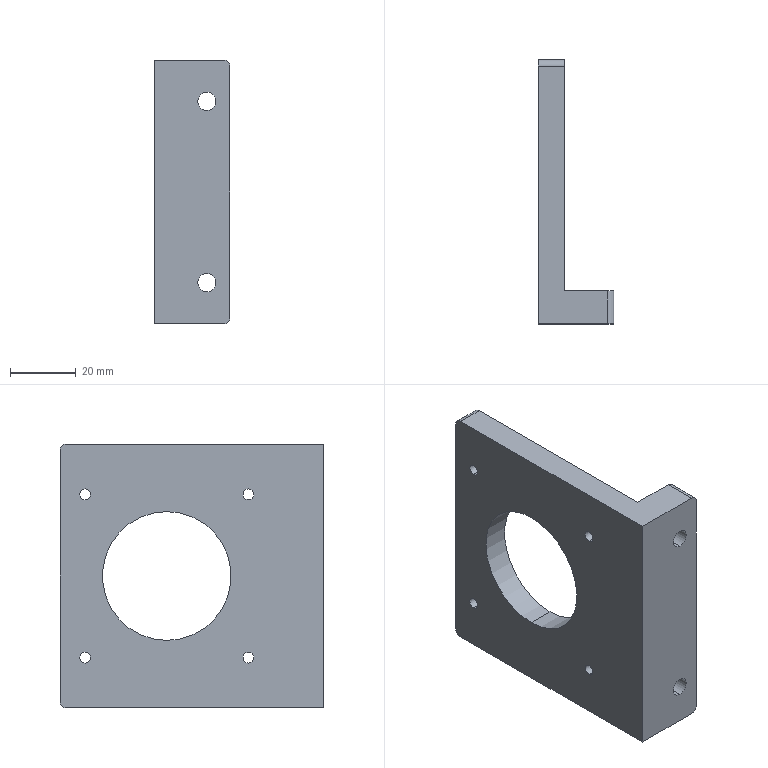Component | SolidWorks | ZHDJ-G003-1 | 1 solid | 32 faces | box 23 x 80 x 80 mm | volume 52239 mm3 | cylinder 22 | plane 10 | commonest cylinder face diameters 3.3 x8 10 x4 5.5 x4 4 x4 39 x2
build123d program:
from build123d import *

# Parameters (mm, degrees)
SKETCH1_W             = 80
SKETCH1_H             = 80
BOSS_EXTRUDE1_DEPTH   = 4
SKETCH2_W             = 80
SKETCH2_H             = 10
BOSS_EXTRUDE2_DEPTH   = 15
SKETCH3_R             = 19.5
CUT_EXTRUDE1_DEPTH    = 20
FILLET1_R             = 2
M4_TAPPED_HOLE1_D     = 3.3
M4_TAPPED_HOLE1_DEPTH = 11.5
M4_TAPPED_HOLE1_TIP   = 0.9914


with BuildPart() as part:
    # Sketch1 → Boss-Extrude1 (new, symmetric)
    with BuildSketch(Plane(origin=(0, 0, 0), x_dir=(0, 0, -1), z_dir=(1, 0, 0))):
        Rectangle(SKETCH1_W, SKETCH1_H)
    extrude(amount=BOSS_EXTRUDE1_DEPTH, both=True)

    # Sketch2 → Boss-Extrude2 (add)
    with BuildSketch(Plane(origin=(4, 0, 0), x_dir=(0, 0, -1), z_dir=(1, 0, 0))):
        with Locations((0, 35)):
            Rectangle(SKETCH2_W, SKETCH2_H)
    extrude(amount=BOSS_EXTRUDE2_DEPTH)

    # Sketch3 → Cut-Extrude1 (cut)
    with BuildSketch(Plane.ZY.offset(4)):
        with Locations((0, -7.641)):
            Circle(SKETCH3_R)
    extrude(amount=-CUT_EXTRUDE1_DEPTH, mode=Mode.SUBTRACT)

    # Fillet1
    fillet1_edges = [part.edges().sort_by_distance(p)[0] for p in [
        (19, 35, 40),
        (19, 35, -40),
        (0, -40, -40),
        (0, -40, 40),
    ]]
    fillet(fillet1_edges, radius=FILLET1_R)

    # Sketch4 → Hole Size _According to_ Type 1 of Hexag (revolve, cut)
    with BuildSketch(Plane(origin=(12, 30, -27.5), x_dir=(0, 0, -1), z_dir=(1, 0, 0))):
        Polygon((0, 0), (0, 15.652), (2.75, 14), (2.75, 5.7), (5, 5.7), (5, 0), align=None)
    hole_size_according_to_type_1_of_hexag = revolve(axis=Axis((12, 23.65, -27.5), (0, 1, 0)), mode=Mode.SUBTRACT)

    # Mirror1: Hole Size _According to_ Type 1 of Hexag across plane
    add(hole_size_according_to_type_1_of_hexag.mirror(Plane.XY), mode=Mode.SUBTRACT)

    # M4 Tapped Hole1
    with Locations(Plane(origin=(4, 17.108, 24.749), x_dir=(0, 0, 1), z_dir=(1, 0, 0))):
        with Locations((0, 0), (-49.497, 0), (-49.497, 49.497), (0, 49.497)):
            Hole(M4_TAPPED_HOLE1_D / 2, depth=M4_TAPPED_HOLE1_DEPTH)
            with Locations((0, 0, -(M4_TAPPED_HOLE1_DEPTH + M4_TAPPED_HOLE1_TIP / 2))):  # 118° drill point
                Cone(0, M4_TAPPED_HOLE1_D / 2, M4_TAPPED_HOLE1_TIP, mode=Mode.SUBTRACT)


solid = part.part

# Placed as in the assembly
solid = solid.moved(Location((-10, -107.5, 124.987), (180, 0, 0)))
STEP:
#1=COLOUR_RGB('',0.7922,0.8196,0.9333);
#2=FILL_AREA_STYLE_COLOUR('',#1);
#3=FILL_AREA_STYLE('',(#2));
#4=SURFACE_STYLE_FILL_AREA(#3);
#5=SURFACE_SIDE_STYLE('',(#4));
#6=SURFACE_STYLE_USAGE(.BOTH.,#5);
#7=PRESENTATION_STYLE_ASSIGNMENT((#6));
#8=CARTESIAN_POINT('',(-0.5512,-4.906,3.881));
#9=VERTEX_POINT('',#8);
#10=CARTESIAN_POINT('',(-0.5512,-4.906,4.011));
#11=VERTEX_POINT('',#10);
#12=CARTESIAN_POINT('',(-0.5512,-4.906,3.946));
#13=DIRECTION('',(1.,-0.,-0.));
#14=DIRECTION('',(0.,0.,1.));
#15=AXIS2_PLACEMENT_3D('',#12,#13,#14);
#16=CIRCLE('',#15,0.06496);
#17=EDGE_CURVE('',#9,#11,#16,.T.);
#18=ORIENTED_EDGE('',*,*,#17,.F.);
#19=CARTESIAN_POINT('',(-0.2362,-4.906,3.881));
#20=VERTEX_POINT('',#19);
#21=CARTESIAN_POINT('',(-0.2362,-4.906,3.881));
#22=DIRECTION('',(1.,-0.,-0.));
#23=VECTOR('',#22,39.37);
#24=LINE('',#21,#23);
#25=EDGE_CURVE('',#9,#20,#24,.T.);
#26=ORIENTED_EDGE('',*,*,#25,.T.);
#27=CARTESIAN_POINT('',(-0.2362,-4.906,4.011));
#28=VERTEX_POINT('',#27);
#29=CARTESIAN_POINT('',(-0.2362,-4.906,3.946));
#30=DIRECTION('',(1.,-0.,-0.));
#31=DIRECTION('',(0.,0.,1.));
#32=AXIS2_PLACEMENT_3D('',#29,#30,#31);
#33=CIRCLE('',#32,0.06496);
#34=EDGE_CURVE('',#20,#28,#33,.T.);
#35=ORIENTED_EDGE('',*,*,#34,.T.);
#36=CARTESIAN_POINT('',(-0.2362,-4.906,4.011));
#37=DIRECTION('',(1.,-0.,-0.));
#38=VECTOR('',#37,39.37);
#39=LINE('',#36,#38);
#40=EDGE_CURVE('',#11,#28,#39,.T.);
#41=ORIENTED_EDGE('',*,*,#40,.F.);
#42=EDGE_LOOP('',(#18,#26,#35,#41));
#43=FACE_OUTER_BOUND('',#42,.T.);
#44=CARTESIAN_POINT('',(-0.2362,-4.906,3.946));
#45=DIRECTION('',(1.,-0.,-0.));
#46=DIRECTION('',(0.,0.,1.));
#47=AXIS2_PLACEMENT_3D('',#44,#45,#46);
#48=CYLINDRICAL_SURFACE('',#47,0.06496);
#49=ADVANCED_FACE('',(#43),#48,.F.);
#50=CARTESIAN_POINT('',(-0.5512,-4.906,5.83));
#51=VERTEX_POINT('',#50);
#52=CARTESIAN_POINT('',(-0.5512,-4.906,5.96));
#53=VERTEX_POINT('',#52);
#54=CARTESIAN_POINT('',(-0.5512,-4.906,5.895));
#55=DIRECTION('',(1.,-0.,-0.));
#56=DIRECTION('',(0.,0.,1.));
#57=AXIS2_PLACEMENT_3D('',#54,#55,#56);
#58=CIRCLE('',#57,0.06496);
#59=EDGE_CURVE('',#51,#53,#58,.T.);
#60=ORIENTED_EDGE('',*,*,#59,.F.);
#61=CARTESIAN_POINT('',(-0.2362,-4.906,5.83));
#62=VERTEX_POINT('',#61);
#63=CARTESIAN_POINT('',(-0.2362,-4.906,5.83));
#64=DIRECTION('',(1.,-0.,-0.));
#65=VECTOR('',#64,39.37);
#66=LINE('',#63,#65);
#67=EDGE_CURVE('',#51,#62,#66,.T.);
#68=ORIENTED_EDGE('',*,*,#67,.T.);
#69=CARTESIAN_POINT('',(-0.2362,-4.906,5.96));
#70=VERTEX_POINT('',#69);
#71=CARTESIAN_POINT('',(-0.2362,-4.906,5.895));
#72=DIRECTION('',(1.,-0.,-0.));
#73=DIRECTION('',(0.,0.,1.));
#74=AXIS2_PLACEMENT_3D('',#71,#72,#73);
#75=CIRCLE('',#74,0.06496);
#76=EDGE_CURVE('',#62,#70,#75,.T.);
#77=ORIENTED_EDGE('',*,*,#76,.T.);
#78=CARTESIAN_POINT('',(-0.2362,-4.906,5.96));
#79=DIRECTION('',(1.,-0.,-0.));
#80=VECTOR('',#79,39.37);
#81=LINE('',#78,#80);
#82=EDGE_CURVE('',#53,#70,#81,.T.);
#83=ORIENTED_EDGE('',*,*,#82,.F.);
#84=EDGE_LOOP('',(#60,#68,#77,#83));
#85=FACE_OUTER_BOUND('',#84,.T.);
#86=CARTESIAN_POINT('',(-0.2362,-4.906,5.895));
#87=DIRECTION('',(1.,-0.,-0.));
#88=DIRECTION('',(0.,0.,1.));
#89=AXIS2_PLACEMENT_3D('',#86,#87,#88);
#90=CYLINDRICAL_SURFACE('',#89,0.06496);
#91=ADVANCED_FACE('',(#85),#90,.F.);
#92=CARTESIAN_POINT('',(-0.5512,-2.957,5.83));
#93=VERTEX_POINT('',#92);
#94=CARTESIAN_POINT('',(-0.5512,-2.957,5.96));
#95=VERTEX_POINT('',#94);
#96=CARTESIAN_POINT('',(-0.5512,-2.957,5.895));
#97=DIRECTION('',(1.,-0.,-0.));
#98=DIRECTION('',(0.,0.,1.));
#99=AXIS2_PLACEMENT_3D('',#96,#97,#98);
#100=CIRCLE('',#99,0.06496);
#101=EDGE_CURVE('',#93,#95,#100,.T.);
#102=ORIENTED_EDGE('',*,*,#101,.F.);
#103=CARTESIAN_POINT('',(-0.2362,-2.957,5.83));
#104=VERTEX_POINT('',#103);
#105=CARTESIAN_POINT('',(-0.2362,-2.957,5.83));
#106=DIRECTION('',(1.,-0.,-0.));
#107=VECTOR('',#106,39.37);
#108=LINE('',#105,#107);
#109=EDGE_CURVE('',#93,#104,#108,.T.);
#110=ORIENTED_EDGE('',*,*,#109,.T.);
#111=CARTESIAN_POINT('',(-0.2362,-2.957,5.96));
#112=VERTEX_POINT('',#111);
#113=CARTESIAN_POINT('',(-0.2362,-2.957,5.895));
#114=DIRECTION('',(1.,-0.,-0.));
#115=DIRECTION('',(0.,0.,1.));
#116=AXIS2_PLACEMENT_3D('',#113,#114,#115);
#117=CIRCLE('',#116,0.06496);
#118=EDGE_CURVE('',#104,#112,#117,.T.);
#119=ORIENTED_EDGE('',*,*,#118,.T.);
#120=CARTESIAN_POINT('',(-0.2362,-2.957,5.96));
#121=DIRECTION('',(1.,-0.,-0.));
#122=VECTOR('',#121,39.37);
#123=LINE('',#120,#122);
#124=EDGE_CURVE('',#95,#112,#123,.T.);
#125=ORIENTED_EDGE('',*,*,#124,.F.);
#126=EDGE_LOOP('',(#102,#110,#119,#125));
#127=FACE_OUTER_BOUND('',#126,.T.);
#128=CARTESIAN_POINT('',(-0.2362,-2.957,5.895));
#129=DIRECTION('',(1.,-0.,-0.));
#130=DIRECTION('',(0.,0.,1.));
#131=AXIS2_PLACEMENT_3D('',#128,#129,#130);
#132=CYLINDRICAL_SURFACE('',#131,0.06496);
#133=ADVANCED_FACE('',(#127),#132,.F.);
#134=CARTESIAN_POINT('',(-0.5512,-2.957,3.881));
#135=VERTEX_POINT('',#134);
#136=CARTESIAN_POINT('',(-0.5512,-2.957,4.011));
#137=VERTEX_POINT('',#136);
#138=CARTESIAN_POINT('',(-0.5512,-2.957,3.946));
#139=DIRECTION('',(1.,-0.,-0.));
#140=DIRECTION('',(0.,0.,1.));
#141=AXIS2_PLACEMENT_3D('',#138,#139,#140);
#142=CIRCLE('',#141,0.06496);
#143=EDGE_CURVE('',#135,#137,#142,.T.);
#144=ORIENTED_EDGE('',*,*,#143,.F.);
#145=CARTESIAN_POINT('',(-0.2362,-2.957,3.881));
#146=VERTEX_POINT('',#145);
#147=CARTESIAN_POINT('',(-0.2362,-2.957,3.881));
#148=DIRECTION('',(1.,-0.,-0.));
#149=VECTOR('',#148,39.37);
#150=LINE('',#147,#149);
#151=EDGE_CURVE('',#135,#146,#150,.T.);
#152=ORIENTED_EDGE('',*,*,#151,.T.);
#153=CARTESIAN_POINT('',(-0.2362,-2.957,4.011));
#154=VERTEX_POINT('',#153);
#155=CARTESIAN_POINT('',(-0.2362,-2.957,3.946));
#156=DIRECTION('',(1.,-0.,-0.));
#157=DIRECTION('',(0.,0.,1.));
#158=AXIS2_PLACEMENT_3D('',#155,#156,#157);
#159=CIRCLE('',#158,0.06496);
#160=EDGE_CURVE('',#146,#154,#159,.T.);
#161=ORIENTED_EDGE('',*,*,#160,.T.);
#162=CARTESIAN_POINT('',(-0.2362,-2.957,4.011));
#163=DIRECTION('',(1.,-0.,-0.));
#164=VECTOR('',#163,39.37);
#165=LINE('',#162,#164);
#166=EDGE_CURVE('',#137,#154,#165,.T.);
#167=ORIENTED_EDGE('',*,*,#166,.F.);
#168=EDGE_LOOP('',(#144,#152,#161,#167));
#169=FACE_OUTER_BOUND('',#168,.T.);
#170=CARTESIAN_POINT('',(-0.2362,-2.957,3.946));
#171=DIRECTION('',(1.,-0.,-0.));
#172=DIRECTION('',(0.,0.,1.));
#173=AXIS2_PLACEMENT_3D('',#170,#171,#172);
#174=CYLINDRICAL_SURFACE('',#173,0.06496);
#175=ADVANCED_FACE('',(#169),#174,.F.);
#176=CARTESIAN_POINT('',(0.07874,-5.638,3.641));
#177=VERTEX_POINT('',#176);
#178=CARTESIAN_POINT('',(0.07874,-5.638,4.035));
#179=VERTEX_POINT('',#178);
#180=CARTESIAN_POINT('',(0.07874,-5.638,3.838));
#181=DIRECTION('',(0.,1.,0.));
#182=DIRECTION('',(0.,0.,1.));
#183=AXIS2_PLACEMENT_3D('',#180,#181,#182);
#184=CIRCLE('',#183,0.1969);
#185=EDGE_CURVE('',#177,#179,#184,.T.);
#186=ORIENTED_EDGE('',*,*,#185,.F.);
#187=CARTESIAN_POINT('',(0.07874,-5.413,3.641));
#188=VERTEX_POINT('',#187);
#189=CARTESIAN_POINT('',(0.07874,-5.413,3.641));
#190=DIRECTION('',(0.,1.,0.));
#191=VECTOR('',#190,39.37);
#192=LINE('',#189,#191);
#193=EDGE_CURVE('',#177,#188,#192,.T.);
#194=ORIENTED_EDGE('',*,*,#193,.T.);
#195=CARTESIAN_POINT('',(0.07874,-5.413,4.035));
#196=VERTEX_POINT('',#195);
#197=CARTESIAN_POINT('',(0.07874,-5.413,3.838));
#198=DIRECTION('',(0.,1.,0.));
#199=DIRECTION('',(0.,0.,1.));
#200=AXIS2_PLACEMENT_3D('',#197,#198,#199);
#201=CIRCLE('',#200,0.1969);
#202=EDGE_CURVE('',#188,#196,#201,.T.);
#203=ORIENTED_EDGE('',*,*,#202,.T.);
#204=CARTESIAN_POINT('',(0.07874,-5.413,4.035));
#205=DIRECTION('',(0.,1.,0.));
#206=VECTOR('',#205,39.37);
#207=LINE('',#204,#206);
#208=EDGE_CURVE('',#179,#196,#207,.T.);
#209=ORIENTED_EDGE('',*,*,#208,.F.);
#210=EDGE_LOOP('',(#186,#194,#203,#209));
#211=FACE_OUTER_BOUND('',#210,.T.);
#212=CARTESIAN_POINT('',(0.07874,-5.413,3.838));
#213=DIRECTION('',(0.,1.,0.));
#214=DIRECTION('',(0.,0.,1.));
#215=AXIS2_PLACEMENT_3D('',#212,#213,#214);
#216=CYLINDRICAL_SURFACE('',#215,0.1969);
#217=ADVANCED_FACE('',(#211),#216,.F.);
#218=CARTESIAN_POINT('',(0.07874,-5.807,3.73));
#219=VERTEX_POINT('',#218);
#220=CARTESIAN_POINT('',(0.07874,-5.807,3.946));
#221=VERTEX_POINT('',#220);
#222=CARTESIAN_POINT('',(0.07874,-5.807,3.838));
#223=DIRECTION('',(0.,1.,0.));
#224=DIRECTION('',(0.,0.,1.));
#225=AXIS2_PLACEMENT_3D('',#222,#223,#224);
#226=CIRCLE('',#225,0.1083);
#227=EDGE_CURVE('',#219,#221,#226,.T.);
#228=ORIENTED_EDGE('',*,*,#227,.F.);
#229=CARTESIAN_POINT('',(0.07874,-5.638,3.73));
#230=VERTEX_POINT('',#229);
#231=CARTESIAN_POINT('',(0.07874,-5.413,3.73));
#232=DIRECTION('',(0.,1.,0.));
#233=VECTOR('',#232,39.37);
#234=LINE('',#231,#233);
#235=EDGE_CURVE('',#219,#230,#234,.T.);
#236=ORIENTED_EDGE('',*,*,#235,.T.);
#237=CARTESIAN_POINT('',(0.07874,-5.638,3.946));
#238=VERTEX_POINT('',#237);
#239=CARTESIAN_POINT('',(0.07874,-5.638,3.838));
#240=DIRECTION('',(0.,1.,0.));
#241=DIRECTION('',(0.,0.,1.));
#242=AXIS2_PLACEMENT_3D('',#239,#240,#241);
#243=CIRCLE('',#242,0.1083);
#244=EDGE_CURVE('',#230,#238,#243,.T.);
#245=ORIENTED_EDGE('',*,*,#244,.T.);
#246=CARTESIAN_POINT('',(0.07874,-5.413,3.946));
#247=DIRECTION('',(0.,1.,0.));
#248=VECTOR('',#247,39.37);
#249=LINE('',#246,#248);
#250=EDGE_CURVE('',#221,#238,#249,.T.);
#251=ORIENTED_EDGE('',*,*,#250,.F.);
#252=EDGE_LOOP('',(#228,#236,#245,#251));
#253=FACE_OUTER_BOUND('',#252,.T.);
#254=CARTESIAN_POINT('',(0.07874,-5.413,3.838));
#255=DIRECTION('',(0.,1.,0.));
#256=DIRECTION('',(0.,0.,1.));
#257=AXIS2_PLACEMENT_3D('',#254,#255,#256);
#258=CYLINDRICAL_SURFACE('',#257,0.1083);
#259=ADVANCED_FACE('',(#253),#258,.F.);
#260=CARTESIAN_POINT('',(0.07874,-5.638,5.807));
#261=VERTEX_POINT('',#260);
#262=CARTESIAN_POINT('',(0.07874,-5.638,6.2));
#263=VERTEX_POINT('',#262);
#264=CARTESIAN_POINT('',(0.07874,-5.638,6.003));
#265=DIRECTION('',(0.,1.,0.));
#266=DIRECTION('',(0.,0.,1.));
#267=AXIS2_PLACEMENT_3D('',#264,#265,#266);
#268=CIRCLE('',#267,0.1969);
#269=EDGE_CURVE('',#261,#263,#268,.T.);
#270=ORIENTED_EDGE('',*,*,#269,.F.);
#271=CARTESIAN_POINT('',(0.07874,-5.413,5.807));
#272=VERTEX_POINT('',#271);
#273=CARTESIAN_POINT('',(0.07874,-5.413,5.807));
#274=DIRECTION('',(0.,1.,0.));
#275=VECTOR('',#274,39.37);
#276=LINE('',#273,#275);
#277=EDGE_CURVE('',#261,#272,#276,.T.);
#278=ORIENTED_EDGE('',*,*,#277,.T.);
#279=CARTESIAN_POINT('',(0.07874,-5.413,6.2));
#280=VERTEX_POINT('',#279);
#281=CARTESIAN_POINT('',(0.07874,-5.413,6.003));
#282=DIRECTION('',(0.,1.,0.));
#283=DIRECTION('',(0.,0.,1.));
#284=AXIS2_PLACEMENT_3D('',#281,#282,#283);
#285=CIRCLE('',#284,0.1969);
#286=EDGE_CURVE('',#272,#280,#285,.T.);
#287=ORIENTED_EDGE('',*,*,#286,.T.);
#288=CARTESIAN_POINT('',(0.07874,-5.413,6.2));
#289=DIRECTION('',(0.,1.,0.));
#290=VECTOR('',#289,39.37);
#291=LINE('',#288,#290);
#292=EDGE_CURVE('',#263,#280,#291,.T.);
#293=ORIENTED_EDGE('',*,*,#292,.F.);
#294=EDGE_LOOP('',(#270,#278,#287,#293));
#295=FACE_OUTER_BOUND('',#294,.T.);
#296=CARTESIAN_POINT('',(0.07874,-5.413,6.003));
#297=DIRECTION('',(0.,1.,0.));
#298=DIRECTION('',(0.,0.,1.));
#299=AXIS2_PLACEMENT_3D('',#296,#297,#298);
#300=CYLINDRICAL_SURFACE('',#299,0.1969);
#301=ADVANCED_FACE('',(#295),#300,.F.);
#302=CARTESIAN_POINT('',(0.07874,-5.807,5.895));
#303=VERTEX_POINT('',#302);
#304=CARTESIAN_POINT('',(0.07874,-5.807,6.112));
#305=VERTEX_POINT('',#304);
#306=CARTESIAN_POINT('',(0.07874,-5.807,6.003));
#307=DIRECTION('',(0.,1.,0.));
#308=DIRECTION('',(0.,0.,1.));
#309=AXIS2_PLACEMENT_3D('',#306,#307,#308);
#310=CIRCLE('',#309,0.1083);
#311=EDGE_CURVE('',#303,#305,#310,.T.);
#312=ORIENTED_EDGE('',*,*,#311,.F.);
#313=CARTESIAN_POINT('',(0.07874,-5.638,5.895));
#314=VERTEX_POINT('',#313);
#315=CARTESIAN_POINT('',(0.07874,-5.413,5.895));
#316=DIRECTION('',(0.,1.,0.));
#317=VECTOR('',#316,39.37);
#318=LINE('',#315,#317);
#319=EDGE_CURVE('',#303,#314,#318,.T.);
#320=ORIENTED_EDGE('',*,*,#319,.T.);
#321=CARTESIAN_POINT('',(0.07874,-5.638,6.112));
#322=VERTEX_POINT('',#321);
#323=CARTESIAN_POINT('',(0.07874,-5.638,6.003));
#324=DIRECTION('',(0.,1.,0.));
#325=DIRECTION('',(0.,0.,1.));
#326=AXIS2_PLACEMENT_3D('',#323,#324,#325);
#327=CIRCLE('',#326,0.1083);
#328=EDGE_CURVE('',#314,#322,#327,.T.);
#329=ORIENTED_EDGE('',*,*,#328,.T.);
#330=CARTESIAN_POINT('',(0.07874,-5.413,6.112));
#331=DIRECTION('',(0.,1.,0.));
#332=VECTOR('',#331,39.37);
#333=LINE('',#330,#332);
#334=EDGE_CURVE('',#305,#322,#333,.T.);
#335=ORIENTED_EDGE('',*,*,#334,.F.);
#336=EDGE_LOOP('',(#312,#320,#329,#335));
#337=FACE_OUTER_BOUND('',#336,.T.);
#338=CARTESIAN_POINT('',(0.07874,-5.413,6.003));
#339=DIRECTION('',(0.,1.,0.));
#340=DIRECTION('',(0.,0.,1.));
#341=AXIS2_PLACEMENT_3D('',#338,#339,#340);
#342=CYLINDRICAL_SURFACE('',#341,0.1083);
#343=ADVANCED_FACE('',(#337),#342,.F.);
#344=CARTESIAN_POINT('',(-0.2362,-3.931,4.153));
#345=VERTEX_POINT('',#344);
#346=CARTESIAN_POINT('',(-0.2362,-3.931,5.688));
#347=VERTEX_POINT('',#346);
#348=CARTESIAN_POINT('',(-0.2362,-3.931,4.921));
#349=DIRECTION('',(1.,-0.,-0.));
#350=DIRECTION('',(0.,0.,1.));
#351=AXIS2_PLACEMENT_3D('',#348,#349,#350);
#352=CIRCLE('',#351,0.7677);
#353=EDGE_CURVE('',#345,#347,#352,.T.);
#354=ORIENTED_EDGE('',*,*,#353,.T.);
#355=CARTESIAN_POINT('',(-0.5512,-3.931,5.688));
#356=VERTEX_POINT('',#355);
#357=CARTESIAN_POINT('',(0.2362,-3.931,5.688));
#358=DIRECTION('',(-1.,0.,0.));
#359=VECTOR('',#358,39.37);
#360=LINE('',#357,#359);
#361=EDGE_CURVE('',#347,#356,#360,.T.);
#362=ORIENTED_EDGE('',*,*,#361,.T.);
#363=CARTESIAN_POINT('',(-0.5512,-3.931,4.153));
#364=VERTEX_POINT('',#363);
#365=CARTESIAN_POINT('',(-0.5512,-3.931,4.921));
#366=DIRECTION('',(-1.,0.,0.));
#367=DIRECTION('',(0.,0.,-1.));
#368=AXIS2_PLACEMENT_3D('',#365,#366,#367);
#369=CIRCLE('',#368,0.7677);
#370=EDGE_CURVE('',#356,#364,#369,.T.);
#371=ORIENTED_EDGE('',*,*,#370,.T.);
#372=CARTESIAN_POINT('',(0.2362,-3.931,4.153));
#373=DIRECTION('',(-1.,0.,0.));
#374=VECTOR('',#373,39.37);
#375=LINE('',#372,#374);
#376=EDGE_CURVE('',#345,#364,#375,.T.);
#377=ORIENTED_EDGE('',*,*,#376,.F.);
#378=EDGE_LOOP('',(#354,#362,#371,#377));
#379=FACE_OUTER_BOUND('',#378,.T.);
#380=CARTESIAN_POINT('',(0.2362,-3.931,4.921));
#381=DIRECTION('',(-1.,0.,0.));
#382=DIRECTION('',(0.,0.,-1.));
#383=AXIS2_PLACEMENT_3D('',#380,#381,#382);
#384=CYLINDRICAL_SURFACE('',#383,0.7677);
#385=ADVANCED_FACE('',(#379),#384,.F.);
#386=CARTESIAN_POINT('',(0.2756,-5.413,3.346));
#387=VERTEX_POINT('',#386);
#388=CARTESIAN_POINT('',(-0.2362,-5.413,3.346));
#389=VERTEX_POINT('',#388);
#390=CARTESIAN_POINT('',(0.3543,-5.413,3.346));
#391=DIRECTION('',(-1.,0.,0.));
#392=VECTOR('',#391,39.37);
#393=LINE('',#390,#392);
#394=EDGE_CURVE('',#387,#389,#393,.T.);
#395=ORIENTED_EDGE('',*,*,#394,.F.);
#396=CARTESIAN_POINT('',(0.2756,-5.807,3.346));
#397=VERTEX_POINT('',#396);
#398=CARTESIAN_POINT('',(0.2756,-5.807,3.346));
#399=DIRECTION('',(-0.,-1.,0.));
#400=VECTOR('',#399,39.37);
#401=LINE('',#398,#400);
#402=EDGE_CURVE('',#387,#397,#401,.T.);
#403=ORIENTED_EDGE('',*,*,#402,.T.);
#404=CARTESIAN_POINT('',(-0.5512,-5.807,3.346));
#405=VERTEX_POINT('',#404);
#406=CARTESIAN_POINT('',(-0.2362,-5.807,3.346));
#407=DIRECTION('',(-1.,0.,0.));
#408=VECTOR('',#407,39.37);
#409=LINE('',#406,#408);
#410=EDGE_CURVE('',#397,#405,#409,.T.);
#411=ORIENTED_EDGE('',*,*,#410,.T.);
#412=CARTESIAN_POINT('',(-0.5512,-2.736,3.346));
#413=VERTEX_POINT('',#412);
#414=CARTESIAN_POINT('',(-0.5512,-2.657,3.346));
#415=DIRECTION('',(0.,1.,0.));
#416=VECTOR('',#415,39.37);
#417=LINE('',#414,#416);
#418=EDGE_CURVE('',#405,#413,#417,.T.);
#419=ORIENTED_EDGE('',*,*,#418,.T.);
#420=CARTESIAN_POINT('',(-0.2362,-2.736,3.346));
#421=VERTEX_POINT('',#420);
#422=CARTESIAN_POINT('',(-0.2362,-2.736,3.346));
#423=DIRECTION('',(1.,-0.,-0.));
#424=VECTOR('',#423,39.37);
#425=LINE('',#422,#424);
#426=EDGE_CURVE('',#413,#421,#425,.T.);
#427=ORIENTED_EDGE('',*,*,#426,.T.);
#428=CARTESIAN_POINT('',(-0.2362,-2.657,3.346));
#429=DIRECTION('',(0.,1.,0.));
#430=VECTOR('',#429,39.37);
#431=LINE('',#428,#430);
#432=EDGE_CURVE('',#389,#421,#431,.T.);
#433=ORIENTED_EDGE('',*,*,#432,.F.);
#434=EDGE_LOOP('',(#395,#403,#411,#419,#427,#433));
#435=FACE_OUTER_BOUND('',#434,.T.);
#436=CARTESIAN_POINT('',(-0.2362,-2.657,3.346));
#437=DIRECTION('',(0.,0.,1.));
#438=DIRECTION('',(-1.,0.,0.));
#439=AXIS2_PLACEMENT_3D('',#436,#437,#438);
#440=PLANE('',#439);
#441=ADVANCED_FACE('',(#435),#440,.F.);
#442=CARTESIAN_POINT('',(-0.5512,-2.657,3.425));
#443=VERTEX_POINT('',#442);
#444=CARTESIAN_POINT('',(-0.5512,-2.657,6.417));
#445=VERTEX_POINT('',#444);
#446=CARTESIAN_POINT('',(-0.5512,-2.657,6.496));
#447=DIRECTION('',(0.,-0.,1.));
#448=VECTOR('',#447,39.37);
#449=LINE('',#446,#448);
#450=EDGE_CURVE('',#443,#445,#449,.T.);
#451=ORIENTED_EDGE('',*,*,#450,.T.);
#452=CARTESIAN_POINT('',(-0.2362,-2.657,6.417));
#453=VERTEX_POINT('',#452);
#454=CARTESIAN_POINT('',(-0.2362,-2.657,6.417));
#455=DIRECTION('',(1.,-0.,-0.));
#456=VECTOR('',#455,39.37);
#457=LINE('',#454,#456);
#458=EDGE_CURVE('',#445,#453,#457,.T.);
#459=ORIENTED_EDGE('',*,*,#458,.T.);
#460=CARTESIAN_POINT('',(-0.2362,-2.657,3.425));
#461=VERTEX_POINT('',#460);
#462=CARTESIAN_POINT('',(-0.2362,-2.657,6.496));
#463=DIRECTION('',(0.,-0.,1.));
#464=VECTOR('',#463,39.37);
#465=LINE('',#462,#464);
#466=EDGE_CURVE('',#461,#453,#465,.T.);
#467=ORIENTED_EDGE('',*,*,#466,.F.);
#468=CARTESIAN_POINT('',(-0.2362,-2.657,3.425));
#469=DIRECTION('',(-1.,0.,0.));
#470=VECTOR('',#469,39.37);
#471=LINE('',#468,#470);
#472=EDGE_CURVE('',#461,#443,#471,.T.);
#473=ORIENTED_EDGE('',*,*,#472,.T.);
#474=EDGE_LOOP('',(#451,#459,#467,#473));
#475=FACE_OUTER_BOUND('',#474,.T.);
#476=CARTESIAN_POINT('',(-0.2362,-2.657,6.496));
#477=DIRECTION('',(-0.,-1.,-0.));
#478=DIRECTION('',(-0.,0.,-1.));
#479=AXIS2_PLACEMENT_3D('',#476,#477,#478);
#480=PLANE('',#479);
#481=ADVANCED_FACE('',(#475),#480,.F.);
#482=CARTESIAN_POINT('',(0.2756,-5.807,6.496));
#483=VERTEX_POINT('',#482);
#484=CARTESIAN_POINT('',(-0.5512,-5.807,6.496));
#485=VERTEX_POINT('',#484);
#486=CARTESIAN_POINT('',(-0.2362,-5.807,6.496));
#487=DIRECTION('',(-1.,0.,0.));
#488=VECTOR('',#487,39.37);
#489=LINE('',#486,#488);
#490=EDGE_CURVE('',#483,#485,#489,.T.);
#491=ORIENTED_EDGE('',*,*,#490,.F.);
#492=CARTESIAN_POINT('',(0.2756,-5.413,6.496));
#493=VERTEX_POINT('',#492);
#494=CARTESIAN_POINT('',(0.2756,-5.413,6.496));
#495=DIRECTION('',(0.,1.,0.));
#496=VECTOR('',#495,39.37);
#497=LINE('',#494,#496);
#498=EDGE_CURVE('',#483,#493,#497,.T.);
#499=ORIENTED_EDGE('',*,*,#498,.T.);
#500=CARTESIAN_POINT('',(-0.2362,-5.413,6.496));
#501=VERTEX_POINT('',#500);
#502=CARTESIAN_POINT('',(0.3543,-5.413,6.496));
#503=DIRECTION('',(-1.,0.,0.));
#504=VECTOR('',#503,39.37);
#505=LINE('',#502,#504);
#506=EDGE_CURVE('',#493,#501,#505,.T.);
#507=ORIENTED_EDGE('',*,*,#506,.T.);
#508=CARTESIAN_POINT('',(-0.2362,-2.736,6.496));
#509=VERTEX_POINT('',#508);
#510=CARTESIAN_POINT('',(-0.2362,-2.657,6.496));
#511=DIRECTION('',(-0.,-1.,0.));
#512=VECTOR('',#511,39.37);
#513=LINE('',#510,#512);
#514=EDGE_CURVE('',#509,#501,#513,.T.);
#515=ORIENTED_EDGE('',*,*,#514,.F.);
#516=CARTESIAN_POINT('',(-0.5512,-2.736,6.496));
#517=VERTEX_POINT('',#516);
#518=CARTESIAN_POINT('',(-0.2362,-2.736,6.496));
#519=DIRECTION('',(-1.,0.,0.));
#520=VECTOR('',#519,39.37);
#521=LINE('',#518,#520);
#522=EDGE_CURVE('',#509,#517,#521,.T.);
#523=ORIENTED_EDGE('',*,*,#522,.T.);
#524=CARTESIAN_POINT('',(-0.5512,-2.657,6.496));
#525=DIRECTION('',(-0.,-1.,0.));
#526=VECTOR('',#525,39.37);
#527=LINE('',#524,#526);
#528=EDGE_CURVE('',#517,#485,#527,.T.);
#529=ORIENTED_EDGE('',*,*,#528,.T.);
#530=EDGE_LOOP('',(#491,#499,#507,#515,#523,#529));
#531=FACE_OUTER_BOUND('',#530,.T.);
#532=CARTESIAN_POINT('',(-0.2362,-2.657,6.496));
#533=DIRECTION('',(-0.,-0.,-1.));
#534=DIRECTION('',(1.,-0.,-0.));
#535=AXIS2_PLACEMENT_3D('',#532,#533,#534);
#536=PLANE('',#535);
#537=ADVANCED_FACE('',(#531),#536,.F.);
#538=CARTESIAN_POINT('',(0.07874,-5.807,3.838));
#539=DIRECTION('',(0.,1.,0.));
#540=DIRECTION('',(0.,0.,1.));
#541=AXIS2_PLACEMENT_3D('',#538,#539,#540);
#542=CIRCLE('',#541,0.1083);
#543=EDGE_CURVE('',#221,#219,#542,.T.);
#544=ORIENTED_EDGE('',*,*,#543,.T.);
#545=ORIENTED_EDGE('',*,*,#227,.T.);
#546=EDGE_LOOP('',(#544,#545));
#547=FACE_BOUND('',#546,.T.);
#548=CARTESIAN_POINT('',(0.07874,-5.807,6.003));
#549=DIRECTION('',(0.,1.,0.));
#550=DIRECTION('',(0.,0.,1.));
#551=AXIS2_PLACEMENT_3D('',#548,#549,#550);
#552=CIRCLE('',#551,0.1083);
#553=EDGE_CURVE('',#305,#303,#552,.T.);
#554=ORIENTED_EDGE('',*,*,#553,.T.);
#555=ORIENTED_EDGE('',*,*,#311,.T.);
#556=EDGE_LOOP('',(#554,#555));
#557=FACE_BOUND('',#556,.T.);
#558=CARTESIAN_POINT('',(0.3543,-5.807,6.417));
#559=VERTEX_POINT('',#558);
#560=CARTESIAN_POINT('',(0.3543,-5.807,3.425));
#561=VERTEX_POINT('',#560);
#562=CARTESIAN_POINT('',(0.3543,-5.807,3.346));
#563=DIRECTION('',(-0.,0.,-1.));
#564=VECTOR('',#563,39.37);
#565=LINE('',#562,#564);
#566=EDGE_CURVE('',#559,#561,#565,.T.);
#567=ORIENTED_EDGE('',*,*,#566,.F.);
#568=CARTESIAN_POINT('',(0.2756,-5.807,6.417));
#569=DIRECTION('',(-0.,-1.,-0.));
#570=DIRECTION('',(0.,0.,1.));
#571=AXIS2_PLACEMENT_3D('',#568,#569,#570);
#572=CIRCLE('',#571,0.07874);
#573=EDGE_CURVE('',#559,#483,#572,.T.);
#574=ORIENTED_EDGE('',*,*,#573,.T.);
#575=ORIENTED_EDGE('',*,*,#490,.T.);
#576=CARTESIAN_POINT('',(-0.5512,-5.807,6.496));
#577=DIRECTION('',(-0.,0.,-1.));
#578=VECTOR('',#577,39.37);
#579=LINE('',#576,#578);
#580=EDGE_CURVE('',#485,#405,#579,.T.);
#581=ORIENTED_EDGE('',*,*,#580,.T.);
#582=ORIENTED_EDGE('',*,*,#410,.F.);
#583=CARTESIAN_POINT('',(0.2756,-5.807,3.425));
#584=DIRECTION('',(-0.,-1.,-0.));
#585=DIRECTION('',(0.,0.,1.));
#586=AXIS2_PLACEMENT_3D('',#583,#584,#585);
#587=CIRCLE('',#586,0.07874);
#588=EDGE_CURVE('',#397,#561,#587,.T.);
#589=ORIENTED_EDGE('',*,*,#588,.T.);
#590=EDGE_LOOP('',(#567,#574,#575,#581,#582,#589));
#591=FACE_OUTER_BOUND('',#590,.T.);
#592=CARTESIAN_POINT('',(-0.2362,-5.807,6.496));
#593=DIRECTION('',(0.,1.,0.));
#594=DIRECTION('',(0.,-0.,1.));
#595=AXIS2_PLACEMENT_3D('',#592,#593,#594);
#596=PLANE('',#595);
#597=ADVANCED_FACE('',(#547,#557,#591),#596,.F.);
#598=CARTESIAN_POINT('',(-0.2362,-4.906,3.946));
#599=DIRECTION('',(1.,-0.,-0.));
#600=DIRECTION('',(0.,0.,1.));
#601=AXIS2_PLACEMENT_3D('',#598,#599,#600);
#602=CIRCLE('',#601,0.06496);
#603=EDGE_CURVE('',#28,#20,#602,.T.);
#604=ORIENTED_EDGE('',*,*,#603,.F.);
#605=ORIENTED_EDGE('',*,*,#34,.F.);
#606=EDGE_LOOP('',(#604,#605));
#607=FACE_BOUND('',#606,.T.);
#608=CARTESIAN_POINT('',(-0.2362,-4.906,5.895));
#609=DIRECTION('',(1.,-0.,-0.));
#610=DIRECTION('',(0.,0.,1.));
#611=AXIS2_PLACEMENT_3D('',#608,#609,#610);
#612=CIRCLE('',#611,0.06496);
#613=EDGE_CURVE('',#70,#62,#612,.T.);
#614=ORIENTED_EDGE('',*,*,#613,.F.);
#615=ORIENTED_EDGE('',*,*,#76,.F.);
#616=EDGE_LOOP('',(#614,#615));
#617=FACE_BOUND('',#616,.T.);
#618=CARTESIAN_POINT('',(-0.2362,-2.957,5.895));
#619=DIRECTION('',(1.,-0.,-0.));
#620=DIRECTION('',(0.,0.,1.));
#621=AXIS2_PLACEMENT_3D('',#618,#619,#620);
#622=CIRCLE('',#621,0.06496);
#623=EDGE_CURVE('',#112,#104,#622,.T.);
#624=ORIENTED_EDGE('',*,*,#623,.F.);
#625=ORIENTED_EDGE('',*,*,#118,.F.);
#626=EDGE_LOOP('',(#624,#625));
#627=FACE_BOUND('',#626,.T.);
#628=CARTESIAN_POINT('',(-0.2362,-2.957,3.946));
#629=DIRECTION('',(1.,-0.,-0.));
#630=DIRECTION('',(0.,0.,1.));
#631=AXIS2_PLACEMENT_3D('',#628,#629,#630);
#632=CIRCLE('',#631,0.06496);
#633=EDGE_CURVE('',#154,#146,#632,.T.);
#634=ORIENTED_EDGE('',*,*,#633,.F.);
#635=ORIENTED_EDGE('',*,*,#160,.F.);
#636=EDGE_LOOP('',(#634,#635));
#637=FACE_BOUND('',#636,.T.);
#638=ORIENTED_EDGE('',*,*,#353,.F.);
#639=CARTESIAN_POINT('',(-0.2362,-3.931,4.921));
#640=DIRECTION('',(1.,-0.,-0.));
#641=DIRECTION('',(0.,0.,1.));
#642=AXIS2_PLACEMENT_3D('',#639,#640,#641);
#643=CIRCLE('',#642,0.7677);
#644=EDGE_CURVE('',#347,#345,#643,.T.);
#645=ORIENTED_EDGE('',*,*,#644,.F.);
#646=EDGE_LOOP('',(#638,#645));
#647=FACE_BOUND('',#646,.T.);
#648=ORIENTED_EDGE('',*,*,#466,.T.);
#649=CARTESIAN_POINT('',(-0.2362,-2.736,6.417));
#650=DIRECTION('',(1.,-0.,-0.));
#651=DIRECTION('',(0.,0.,1.));
#652=AXIS2_PLACEMENT_3D('',#649,#650,#651);
#653=CIRCLE('',#652,0.07874);
#654=EDGE_CURVE('',#453,#509,#653,.T.);
#655=ORIENTED_EDGE('',*,*,#654,.T.);
#656=ORIENTED_EDGE('',*,*,#514,.T.);
#657=CARTESIAN_POINT('',(-0.2362,-5.413,3.346));
#658=DIRECTION('',(0.,-0.,1.));
#659=VECTOR('',#658,39.37);
#660=LINE('',#657,#659);
#661=EDGE_CURVE('',#389,#501,#660,.T.);
#662=ORIENTED_EDGE('',*,*,#661,.F.);
#663=ORIENTED_EDGE('',*,*,#432,.T.);
#664=CARTESIAN_POINT('',(-0.2362,-2.736,3.425));
#665=DIRECTION('',(1.,-0.,-0.));
#666=DIRECTION('',(0.,0.,1.));
#667=AXIS2_PLACEMENT_3D('',#664,#665,#666);
#668=CIRCLE('',#667,0.07874);
#669=EDGE_CURVE('',#421,#461,#668,.T.);
#670=ORIENTED_EDGE('',*,*,#669,.T.);
#671=EDGE_LOOP('',(#648,#655,#656,#662,#663,#670));
#672=FACE_OUTER_BOUND('',#671,.T.);
#673=CARTESIAN_POINT('',(-0.2362,-4.232,4.921));
#674=DIRECTION('',(1.,-0.,-0.));
#675=DIRECTION('',(0.,0.,1.));
#676=AXIS2_PLACEMENT_3D('',#673,#674,#675);
#677=PLANE('',#676);
#678=ADVANCED_FACE('',(#607,#617,#627,#637,#647,#672),#677,.T.);
#679=CARTESIAN_POINT('',(-0.5512,-4.906,3.946));
#680=DIRECTION('',(1.,-0.,-0.));
#681=DIRECTION('',(0.,0.,1.));
#682=AXIS2_PLACEMENT_3D('',#679,#680,#681);
#683=CIRCLE('',#682,0.06496);
#684=EDGE_CURVE('',#11,#9,#683,.T.);
#685=ORIENTED_EDGE('',*,*,#684,.T.);
#686=ORIENTED_EDGE('',*,*,#17,.T.);
#687=EDGE_LOOP('',(#685,#686));
#688=FACE_BOUND('',#687,.T.);
#689=CARTESIAN_POINT('',(-0.5512,-4.906,5.895));
#690=DIRECTION('',(1.,-0.,-0.));
#691=DIRECTION('',(0.,0.,1.));
#692=AXIS2_PLACEMENT_3D('',#689,#690,#691);
#693=CIRCLE('',#692,0.06496);
#694=EDGE_CURVE('',#53,#51,#693,.T.);
#695=ORIENTED_EDGE('',*,*,#694,.T.);
#696=ORIENTED_EDGE('',*,*,#59,.T.);
#697=EDGE_LOOP('',(#695,#696));
#698=FACE_BOUND('',#697,.T.);
#699=CARTESIAN_POINT('',(-0.5512,-2.957,5.895));
#700=DIRECTION('',(1.,-0.,-0.));
#701=DIRECTION('',(0.,0.,1.));
#702=AXIS2_PLACEMENT_3D('',#699,#700,#701);
#703=CIRCLE('',#702,0.06496);
#704=EDGE_CURVE('',#95,#93,#703,.T.);
#705=ORIENTED_EDGE('',*,*,#704,.T.);
#706=ORIENTED_EDGE('',*,*,#101,.T.);
#707=EDGE_LOOP('',(#705,#706));
#708=FACE_BOUND('',#707,.T.);
#709=CARTESIAN_POINT('',(-0.5512,-2.957,3.946));
#710=DIRECTION('',(1.,-0.,-0.));
#711=DIRECTION('',(0.,0.,1.));
#712=AXIS2_PLACEMENT_3D('',#709,#710,#711);
#713=CIRCLE('',#712,0.06496);
#714=EDGE_CURVE('',#137,#135,#713,.T.);
#715=ORIENTED_EDGE('',*,*,#714,.T.);
#716=ORIENTED_EDGE('',*,*,#143,.T.);
#717=EDGE_LOOP('',(#715,#716));
#718=FACE_BOUND('',#717,.T.);
#719=CARTESIAN_POINT('',(-0.5512,-3.931,4.921));
#720=DIRECTION('',(-1.,0.,0.));
#721=DIRECTION('',(0.,0.,-1.));
#722=AXIS2_PLACEMENT_3D('',#719,#720,#721);
#723=CIRCLE('',#722,0.7677);
#724=EDGE_CURVE('',#364,#356,#723,.T.);
#725=ORIENTED_EDGE('',*,*,#724,.F.);
#726=ORIENTED_EDGE('',*,*,#370,.F.);
#727=EDGE_LOOP('',(#725,#726));
#728=FACE_BOUND('',#727,.T.);
#729=ORIENTED_EDGE('',*,*,#528,.F.);
#730=CARTESIAN_POINT('',(-0.5512,-2.736,6.417));
#731=DIRECTION('',(-1.,0.,0.));
#732=DIRECTION('',(0.,0.,1.));
#733=AXIS2_PLACEMENT_3D('',#730,#731,#732);
#734=CIRCLE('',#733,0.07874);
#735=EDGE_CURVE('',#517,#445,#734,.T.);
#736=ORIENTED_EDGE('',*,*,#735,.T.);
#737=ORIENTED_EDGE('',*,*,#450,.F.);
#738=CARTESIAN_POINT('',(-0.5512,-2.736,3.425));
#739=DIRECTION('',(-1.,0.,0.));
#740=DIRECTION('',(0.,0.,1.));
#741=AXIS2_PLACEMENT_3D('',#738,#739,#740);
#742=CIRCLE('',#741,0.07874);
#743=EDGE_CURVE('',#443,#413,#742,.T.);
#744=ORIENTED_EDGE('',*,*,#743,.T.);
#745=ORIENTED_EDGE('',*,*,#418,.F.);
#746=ORIENTED_EDGE('',*,*,#580,.F.);
#747=EDGE_LOOP('',(#729,#736,#737,#744,#745,#746));
#748=FACE_OUTER_BOUND('',#747,.T.);
#749=CARTESIAN_POINT('',(-0.5512,-4.232,4.921));
#750=DIRECTION('',(1.,-0.,-0.));
#751=DIRECTION('',(0.,0.,1.));
#752=AXIS2_PLACEMENT_3D('',#749,#750,#751);
#753=PLANE('',#752);
#754=ADVANCED_FACE('',(#688,#698,#708,#718,#728,#748),#753,.F.);
#755=CARTESIAN_POINT('',(0.07874,-5.413,3.838));
#756=DIRECTION('',(0.,1.,0.));
#757=DIRECTION('',(0.,0.,1.));
#758=AXIS2_PLACEMENT_3D('',#755,#756,#757);
#759=CIRCLE('',#758,0.1969);
#760=EDGE_CURVE('',#196,#188,#759,.T.);
#761=ORIENTED_EDGE('',*,*,#760,.F.);
#762=ORIENTED_EDGE('',*,*,#202,.F.);
#763=EDGE_LOOP('',(#761,#762));
#764=FACE_BOUND('',#763,.T.);
#765=CARTESIAN_POINT('',(0.07874,-5.413,6.003));
#766=DIRECTION('',(0.,1.,0.));
#767=DIRECTION('',(0.,0.,1.));
#768=AXIS2_PLACEMENT_3D('',#765,#766,#767);
#769=CIRCLE('',#768,0.1969);
#770=EDGE_CURVE('',#280,#272,#769,.T.);
#771=ORIENTED_EDGE('',*,*,#770,.F.);
#772=ORIENTED_EDGE('',*,*,#286,.F.);
#773=EDGE_LOOP('',(#771,#772));
#774=FACE_BOUND('',#773,.T.);
#775=ORIENTED_EDGE('',*,*,#506,.F.);
#776=CARTESIAN_POINT('',(0.3543,-5.413,6.417));
#777=VERTEX_POINT('',#776);
#778=CARTESIAN_POINT('',(0.2756,-5.413,6.417));
#779=DIRECTION('',(0.,1.,0.));
#780=DIRECTION('',(0.,0.,-1.));
#781=AXIS2_PLACEMENT_3D('',#778,#779,#780);
#782=CIRCLE('',#781,0.07874);
#783=EDGE_CURVE('',#493,#777,#782,.T.);
#784=ORIENTED_EDGE('',*,*,#783,.T.);
#785=CARTESIAN_POINT('',(0.3543,-5.413,3.425));
#786=VERTEX_POINT('',#785);
#787=CARTESIAN_POINT('',(0.3543,-5.413,3.346));
#788=DIRECTION('',(0.,-0.,1.));
#789=VECTOR('',#788,39.37);
#790=LINE('',#787,#789);
#791=EDGE_CURVE('',#786,#777,#790,.T.);
#792=ORIENTED_EDGE('',*,*,#791,.F.);
#793=CARTESIAN_POINT('',(0.2756,-5.413,3.425));
#794=DIRECTION('',(0.,1.,0.));
#795=DIRECTION('',(0.,0.,-1.));
#796=AXIS2_PLACEMENT_3D('',#793,#794,#795);
#797=CIRCLE('',#796,0.07874);
#798=EDGE_CURVE('',#786,#387,#797,.T.);
#799=ORIENTED_EDGE('',*,*,#798,.T.);
#800=ORIENTED_EDGE('',*,*,#394,.T.);
#801=ORIENTED_EDGE('',*,*,#661,.T.);
#802=EDGE_LOOP('',(#775,#784,#792,#799,#800,#801));
#803=FACE_OUTER_BOUND('',#802,.T.);
#804=CARTESIAN_POINT('',(0.3543,-5.413,3.346));
#805=DIRECTION('',(-0.,-1.,-0.));
#806=DIRECTION('',(-0.,0.,-1.));
#807=AXIS2_PLACEMENT_3D('',#804,#805,#806);
#808=PLANE('',#807);
#809=ADVANCED_FACE('',(#764,#774,#803),#808,.F.);
#810=ORIENTED_EDGE('',*,*,#791,.T.);
#811=CARTESIAN_POINT('',(0.3543,-5.807,6.417));
#812=DIRECTION('',(-0.,-1.,0.));
#813=VECTOR('',#812,39.37);
#814=LINE('',#811,#813);
#815=EDGE_CURVE('',#777,#559,#814,.T.);
#816=ORIENTED_EDGE('',*,*,#815,.T.);
#817=ORIENTED_EDGE('',*,*,#566,.T.);
#818=CARTESIAN_POINT('',(0.3543,-5.413,3.425));
#819=DIRECTION('',(0.,1.,0.));
#820=VECTOR('',#819,39.37);
#821=LINE('',#818,#820);
#822=EDGE_CURVE('',#561,#786,#821,.T.);
#823=ORIENTED_EDGE('',*,*,#822,.T.);
#824=EDGE_LOOP('',(#810,#816,#817,#823));
#825=FACE_OUTER_BOUND('',#824,.T.);
#826=CARTESIAN_POINT('',(0.3543,-4.232,4.921));
#827=DIRECTION('',(1.,-0.,-0.));
#828=DIRECTION('',(0.,0.,1.));
#829=AXIS2_PLACEMENT_3D('',#826,#827,#828);
#830=PLANE('',#829);
#831=ADVANCED_FACE('',(#825),#830,.T.);
#832=ORIENTED_EDGE('',*,*,#361,.F.);
#833=ORIENTED_EDGE('',*,*,#644,.T.);
#834=ORIENTED_EDGE('',*,*,#376,.T.);
#835=ORIENTED_EDGE('',*,*,#724,.T.);
#836=EDGE_LOOP('',(#832,#833,#834,#835));
#837=FACE_OUTER_BOUND('',#836,.T.);
#838=CARTESIAN_POINT('',(0.2362,-3.931,4.921));
#839=DIRECTION('',(-1.,0.,0.));
#840=DIRECTION('',(0.,0.,-1.));
#841=AXIS2_PLACEMENT_3D('',#838,#839,#840);
#842=CYLINDRICAL_SURFACE('',#841,0.7677);
#843=ADVANCED_FACE('',(#837),#842,.F.);
#844=ORIENTED_EDGE('',*,*,#783,.F.);
#845=ORIENTED_EDGE('',*,*,#498,.F.);
#846=ORIENTED_EDGE('',*,*,#573,.F.);
#847=ORIENTED_EDGE('',*,*,#815,.F.);
#848=EDGE_LOOP('',(#844,#845,#846,#847));
#849=FACE_OUTER_BOUND('',#848,.T.);
#850=CARTESIAN_POINT('',(0.2756,-4.232,6.417));
#851=DIRECTION('',(0.,1.,0.));
#852=DIRECTION('',(0.,0.,1.));
#853=AXIS2_PLACEMENT_3D('',#850,#851,#852);
#854=CYLINDRICAL_SURFACE('',#853,0.07874);
#855=ADVANCED_FACE('',(#849),#854,.T.);
#856=ORIENTED_EDGE('',*,*,#654,.F.);
#857=ORIENTED_EDGE('',*,*,#458,.F.);
#858=ORIENTED_EDGE('',*,*,#735,.F.);
#859=ORIENTED_EDGE('',*,*,#522,.F.);
#860=EDGE_LOOP('',(#856,#857,#858,#859));
#861=FACE_OUTER_BOUND('',#860,.T.);
#862=CARTESIAN_POINT('',(-0.2362,-2.736,6.417));
#863=DIRECTION('',(-1.,0.,0.));
#864=DIRECTION('',(0.,0.,-1.));
#865=AXIS2_PLACEMENT_3D('',#862,#863,#864);
#866=CYLINDRICAL_SURFACE('',#865,0.07874);
#867=ADVANCED_FACE('',(#861),#866,.T.);
#868=ORIENTED_EDGE('',*,*,#588,.F.);
#869=ORIENTED_EDGE('',*,*,#402,.F.);
#870=ORIENTED_EDGE('',*,*,#798,.F.);
#871=ORIENTED_EDGE('',*,*,#822,.F.);
#872=EDGE_LOOP('',(#868,#869,#870,#871));
#873=FACE_OUTER_BOUND('',#872,.T.);
#874=CARTESIAN_POINT('',(0.2756,-4.232,3.425));
#875=DIRECTION('',(-0.,-1.,0.));
#876=DIRECTION('',(0.,0.,-1.));
#877=AXIS2_PLACEMENT_3D('',#874,#875,#876);
#878=CYLINDRICAL_SURFACE('',#877,0.07874);
#879=ADVANCED_FACE('',(#873),#878,.T.);
#880=ORIENTED_EDGE('',*,*,#669,.F.);
#881=ORIENTED_EDGE('',*,*,#426,.F.);
#882=ORIENTED_EDGE('',*,*,#743,.F.);
#883=ORIENTED_EDGE('',*,*,#472,.F.);
#884=EDGE_LOOP('',(#880,#881,#882,#883));
#885=FACE_OUTER_BOUND('',#884,.T.);
#886=CARTESIAN_POINT('',(-0.2362,-2.736,3.425));
#887=DIRECTION('',(-1.,0.,0.));
#888=DIRECTION('',(0.,0.,-1.));
#889=AXIS2_PLACEMENT_3D('',#886,#887,#888);
#890=CYLINDRICAL_SURFACE('',#889,0.07874);
#891=ADVANCED_FACE('',(#885),#890,.T.);
#892=ORIENTED_EDGE('',*,*,#319,.F.);
#893=ORIENTED_EDGE('',*,*,#553,.F.);
#894=ORIENTED_EDGE('',*,*,#334,.T.);
#895=CARTESIAN_POINT('',(0.07874,-5.638,6.003));
#896=DIRECTION('',(0.,1.,0.));
#897=DIRECTION('',(0.,0.,1.));
#898=AXIS2_PLACEMENT_3D('',#895,#896,#897);
#899=CIRCLE('',#898,0.1083);
#900=EDGE_CURVE('',#322,#314,#899,.T.);
#901=ORIENTED_EDGE('',*,*,#900,.T.);
#902=EDGE_LOOP('',(#892,#893,#894,#901));
#903=FACE_OUTER_BOUND('',#902,.T.);
#904=CARTESIAN_POINT('',(0.07874,-5.413,6.003));
#905=DIRECTION('',(0.,1.,0.));
#906=DIRECTION('',(0.,0.,1.));
#907=AXIS2_PLACEMENT_3D('',#904,#905,#906);
#908=CYLINDRICAL_SURFACE('',#907,0.1083);
#909=ADVANCED_FACE('',(#903),#908,.F.);
#910=ORIENTED_EDGE('',*,*,#900,.F.);
#911=ORIENTED_EDGE('',*,*,#328,.F.);
#912=EDGE_LOOP('',(#910,#911));
#913=FACE_BOUND('',#912,.T.);
#914=CARTESIAN_POINT('',(0.07874,-5.638,6.003));
#915=DIRECTION('',(0.,1.,0.));
#916=DIRECTION('',(0.,0.,1.));
#917=AXIS2_PLACEMENT_3D('',#914,#915,#916);
#918=CIRCLE('',#917,0.1969);
#919=EDGE_CURVE('',#263,#261,#918,.T.);
#920=ORIENTED_EDGE('',*,*,#919,.T.);
#921=ORIENTED_EDGE('',*,*,#269,.T.);
#922=EDGE_LOOP('',(#920,#921));
#923=FACE_OUTER_BOUND('',#922,.T.);
#924=CARTESIAN_POINT('',(0.187,-5.638,6.003));
#925=DIRECTION('',(-0.,-1.,0.));
#926=DIRECTION('',(-0.,0.,-1.));
#927=AXIS2_PLACEMENT_3D('',#924,#925,#926);
#928=PLANE('',#927);
#929=ADVANCED_FACE('',(#913,#923),#928,.F.);
#930=ORIENTED_EDGE('',*,*,#277,.F.);
#931=ORIENTED_EDGE('',*,*,#919,.F.);
#932=ORIENTED_EDGE('',*,*,#292,.T.);
#933=ORIENTED_EDGE('',*,*,#770,.T.);
#934=EDGE_LOOP('',(#930,#931,#932,#933));
#935=FACE_OUTER_BOUND('',#934,.T.);
#936=CARTESIAN_POINT('',(0.07874,-5.413,6.003));
#937=DIRECTION('',(0.,1.,0.));
#938=DIRECTION('',(0.,0.,1.));
#939=AXIS2_PLACEMENT_3D('',#936,#937,#938);
#940=CYLINDRICAL_SURFACE('',#939,0.1969);
#941=ADVANCED_FACE('',(#935),#940,.F.);
#942=ORIENTED_EDGE('',*,*,#235,.F.);
#943=ORIENTED_EDGE('',*,*,#543,.F.);
#944=ORIENTED_EDGE('',*,*,#250,.T.);
#945=CARTESIAN_POINT('',(0.07874,-5.638,3.838));
#946=DIRECTION('',(0.,1.,0.));
#947=DIRECTION('',(0.,0.,1.));
#948=AXIS2_PLACEMENT_3D('',#945,#946,#947);
#949=CIRCLE('',#948,0.1083);
#950=EDGE_CURVE('',#238,#230,#949,.T.);
#951=ORIENTED_EDGE('',*,*,#950,.T.);
#952=EDGE_LOOP('',(#942,#943,#944,#951));
#953=FACE_OUTER_BOUND('',#952,.T.);
#954=CARTESIAN_POINT('',(0.07874,-5.413,3.838));
#955=DIRECTION('',(0.,1.,0.));
#956=DIRECTION('',(0.,0.,1.));
#957=AXIS2_PLACEMENT_3D('',#954,#955,#956);
#958=CYLINDRICAL_SURFACE('',#957,0.1083);
#959=ADVANCED_FACE('',(#953),#958,.F.);
#960=ORIENTED_EDGE('',*,*,#950,.F.);
#961=ORIENTED_EDGE('',*,*,#244,.F.);
#962=EDGE_LOOP('',(#960,#961));
#963=FACE_BOUND('',#962,.T.);
#964=CARTESIAN_POINT('',(0.07874,-5.638,3.838));
#965=DIRECTION('',(0.,1.,0.));
#966=DIRECTION('',(0.,0.,1.));
#967=AXIS2_PLACEMENT_3D('',#964,#965,#966);
#968=CIRCLE('',#967,0.1969);
#969=EDGE_CURVE('',#179,#177,#968,.T.);
#970=ORIENTED_EDGE('',*,*,#969,.T.);
#971=ORIENTED_EDGE('',*,*,#185,.T.);
#972=EDGE_LOOP('',(#970,#971));
#973=FACE_OUTER_BOUND('',#972,.T.);
#974=CARTESIAN_POINT('',(0.187,-5.638,3.838));
#975=DIRECTION('',(-0.,-1.,0.));
#976=DIRECTION('',(-0.,0.,-1.));
#977=AXIS2_PLACEMENT_3D('',#974,#975,#976);
#978=PLANE('',#977);
#979=ADVANCED_FACE('',(#963,#973),#978,.F.);
#980=ORIENTED_EDGE('',*,*,#193,.F.);
#981=ORIENTED_EDGE('',*,*,#969,.F.);
#982=ORIENTED_EDGE('',*,*,#208,.T.);
#983=ORIENTED_EDGE('',*,*,#760,.T.);
#984=EDGE_LOOP('',(#980,#981,#982,#983));
#985=FACE_OUTER_BOUND('',#984,.T.);
#986=CARTESIAN_POINT('',(0.07874,-5.413,3.838));
#987=DIRECTION('',(0.,1.,0.));
#988=DIRECTION('',(0.,0.,1.));
#989=AXIS2_PLACEMENT_3D('',#986,#987,#988);
#990=CYLINDRICAL_SURFACE('',#989,0.1969);
#991=ADVANCED_FACE('',(#985),#990,.F.);
#992=ORIENTED_EDGE('',*,*,#151,.F.);
#993=ORIENTED_EDGE('',*,*,#714,.F.);
#994=ORIENTED_EDGE('',*,*,#166,.T.);
#995=ORIENTED_EDGE('',*,*,#633,.T.);
#996=EDGE_LOOP('',(#992,#993,#994,#995));
#997=FACE_OUTER_BOUND('',#996,.T.);
#998=CARTESIAN_POINT('',(-0.2362,-2.957,3.946));
#999=DIRECTION('',(1.,-0.,-0.));
#1000=DIRECTION('',(0.,0.,1.));
#1001=AXIS2_PLACEMENT_3D('',#998,#999,#1000);
#1002=CYLINDRICAL_SURFACE('',#1001,0.06496);
#1003=ADVANCED_FACE('',(#997),#1002,.F.);
#1004=ORIENTED_EDGE('',*,*,#109,.F.);
#1005=ORIENTED_EDGE('',*,*,#704,.F.);
#1006=ORIENTED_EDGE('',*,*,#124,.T.);
#1007=ORIENTED_EDGE('',*,*,#623,.T.);
#1008=EDGE_LOOP('',(#1004,#1005,#1006,#1007));
#1009=FACE_OUTER_BOUND('',#1008,.T.);
#1010=CARTESIAN_POINT('',(-0.2362,-2.957,5.895));
#1011=DIRECTION('',(1.,-0.,-0.));
#1012=DIRECTION('',(0.,0.,1.));
#1013=AXIS2_PLACEMENT_3D('',#1010,#1011,#1012);
#1014=CYLINDRICAL_SURFACE('',#1013,0.06496);
#1015=ADVANCED_FACE('',(#1009),#1014,.F.);
#1016=ORIENTED_EDGE('',*,*,#67,.F.);
#1017=ORIENTED_EDGE('',*,*,#694,.F.);
#1018=ORIENTED_EDGE('',*,*,#82,.T.);
#1019=ORIENTED_EDGE('',*,*,#613,.T.);
#1020=EDGE_LOOP('',(#1016,#1017,#1018,#1019));
#1021=FACE_OUTER_BOUND('',#1020,.T.);
#1022=CARTESIAN_POINT('',(-0.2362,-4.906,5.895));
#1023=DIRECTION('',(1.,-0.,-0.));
#1024=DIRECTION('',(0.,0.,1.));
#1025=AXIS2_PLACEMENT_3D('',#1022,#1023,#1024);
#1026=CYLINDRICAL_SURFACE('',#1025,0.06496);
#1027=ADVANCED_FACE('',(#1021),#1026,.F.);
#1028=ORIENTED_EDGE('',*,*,#25,.F.);
#1029=ORIENTED_EDGE('',*,*,#684,.F.);
#1030=ORIENTED_EDGE('',*,*,#40,.T.);
#1031=ORIENTED_EDGE('',*,*,#603,.T.);
#1032=EDGE_LOOP('',(#1028,#1029,#1030,#1031));
#1033=FACE_OUTER_BOUND('',#1032,.T.);
#1034=CARTESIAN_POINT('',(-0.2362,-4.906,3.946));
#1035=DIRECTION('',(1.,-0.,-0.));
#1036=DIRECTION('',(0.,0.,1.));
#1037=AXIS2_PLACEMENT_3D('',#1034,#1035,#1036);
#1038=CYLINDRICAL_SURFACE('',#1037,0.06496);
#1039=ADVANCED_FACE('',(#1033),#1038,.F.);
#1040=CLOSED_SHELL('',(#49,#91,#133,#175,#217,#259,#301,#343,#385,#441,#481,#537,#597,#678,#754,#809,#831,#843,#855,#867,#879,#891,#909,#929,#941,#959,#979,#991,#1003,#1015,#1027,#1039));
#1041=MANIFOLD_SOLID_BREP('',#1040);
#1042=STYLED_ITEM('',(#7),#1041);
#1043=(LENGTH_UNIT()NAMED_UNIT(*)SI_UNIT($,.METRE.));
#1044=LENGTH_MEASURE_WITH_UNIT(LENGTH_MEASURE(0.0254),#1043);
#1045=DIMENSIONAL_EXPONENTS(1.,0.,0.,0.,0.,0.,0.);
#1046=(CONVERSION_BASED_UNIT('',#1044)LENGTH_UNIT()NAMED_UNIT(#1045));
#1047=UNCERTAINTY_MEASURE_WITH_UNIT(LENGTH_MEASURE(0.00001),#1046,'','');
#1048=(NAMED_UNIT(*)PLANE_ANGLE_UNIT()SI_UNIT($,.RADIAN.));
#1049=(NAMED_UNIT(*)SI_UNIT($,.STERADIAN.)SOLID_ANGLE_UNIT());
#1050=(GEOMETRIC_REPRESENTATION_CONTEXT(3)GLOBAL_UNCERTAINTY_ASSIGNED_CONTEXT((#1047))GLOBAL_UNIT_ASSIGNED_CONTEXT((#1046,#1048,#1049))REPRESENTATION_CONTEXT('',''));
#1051=MECHANICAL_DESIGN_GEOMETRIC_PRESENTATION_REPRESENTATION('',(#1042),#1050);
#1052=CARTESIAN_POINT('',(0.,0.,0.));
#1053=DIRECTION('',(0.,0.,1.));
#1054=DIRECTION('',(1.,0.,0.));
#1055=AXIS2_PLACEMENT_3D('',#1052,#1053,#1054);
#1056=(LENGTH_UNIT()NAMED_UNIT(*)SI_UNIT($,.METRE.));
#1057=LENGTH_MEASURE_WITH_UNIT(LENGTH_MEASURE(0.0254),#1056);
#1058=DIMENSIONAL_EXPONENTS(1.,0.,0.,0.,0.,0.,0.);
#1059=(CONVERSION_BASED_UNIT('',#1057)LENGTH_UNIT()NAMED_UNIT(#1058));
#1060=UNCERTAINTY_MEASURE_WITH_UNIT(LENGTH_MEASURE(0.00001),#1059,'','');
#1061=(NAMED_UNIT(*)PLANE_ANGLE_UNIT()SI_UNIT($,.RADIAN.));
#1062=(NAMED_UNIT(*)SI_UNIT($,.STERADIAN.)SOLID_ANGLE_UNIT());
#1063=(GEOMETRIC_REPRESENTATION_CONTEXT(3)GLOBAL_UNCERTAINTY_ASSIGNED_CONTEXT((#1060))GLOBAL_UNIT_ASSIGNED_CONTEXT((#1059,#1061,#1062))REPRESENTATION_CONTEXT('',''));
#1064=ADVANCED_BREP_SHAPE_REPRESENTATION('',(#1041,#1055),#1063);
#1065=PRESENTATION_LAYER_ASSIGNMENT('','',(#1042));